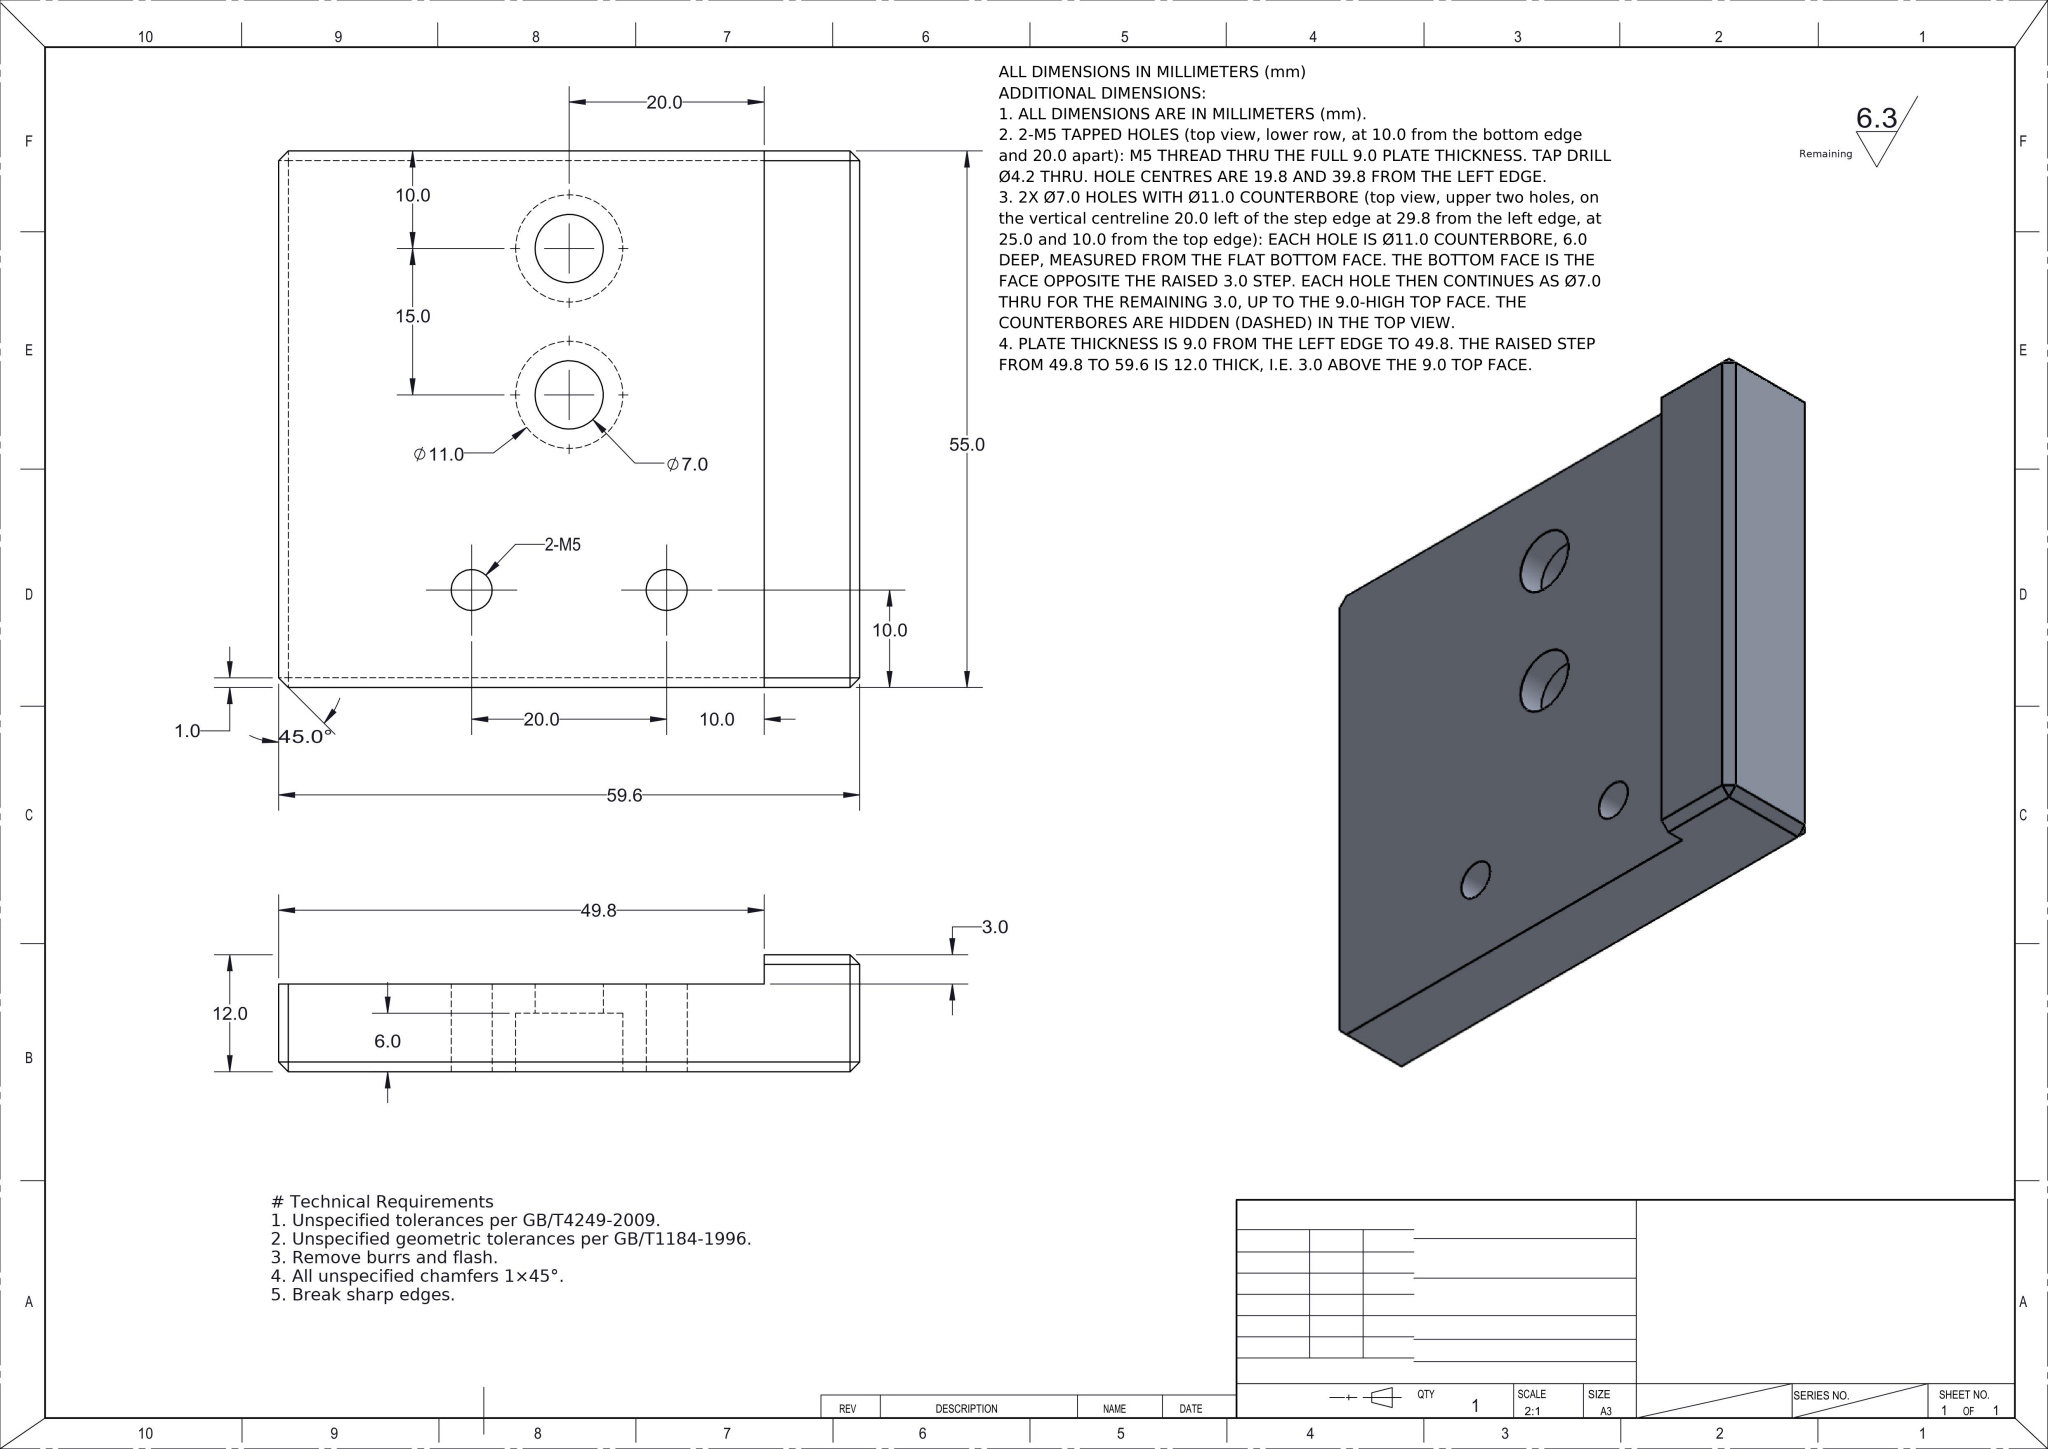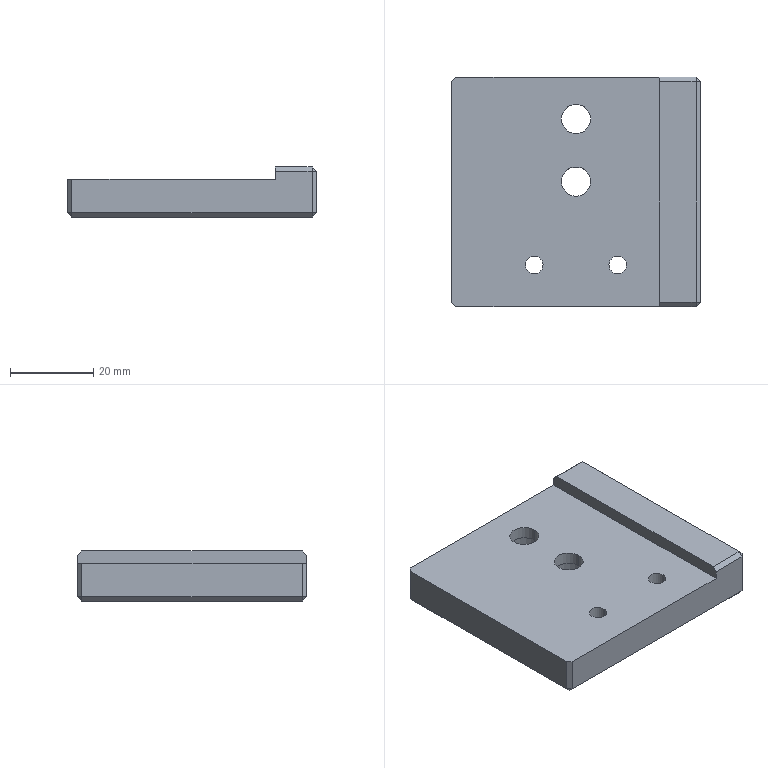Part | NX | mm | Notched Random Bore Plate | 1 solid | 39 faces | box 59.6 x 55 x 12 mm | volume 29329 mm3 | plane 27 | cylinder 12 | commonest cylinder face diameters 11 x4 7 x4 4.2 x4